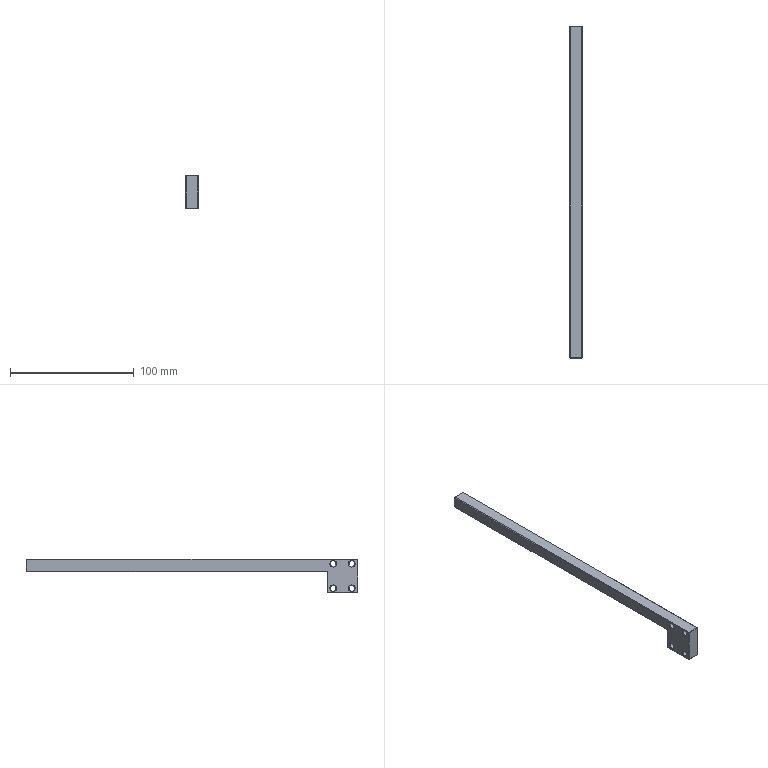Component | SolidWorks | BearingHousingAssembly-1_CylinderJaw1-1 | 1 solid | 60 faces | box 10 x 268 x 27 mm | volume 30124 mm3 | plane 32 | cone 18 | cylinder 10 | commonest cylinder face diameters 4.5 x8 3.3 x2 | material Plain Carbon Steel
build123d program:
from build123d import *

# Parameters (mm, degrees)
BOSS_EXTRUDE1_DEPTH            = 5
F_4_5_4_5_DIAMETER_HOLE1_D     = 4.5
F_4_5_4_5_DIAMETER_HOLE1_DEPTH = 50
F_4_5_4_5_DIAMETER_HOLE1_TIP   = 1.352
CHAMFER1_SIZE                  = 0.5
M4_TAPPED_HOLE1_D              = 3.3
M4_TAPPED_HOLE1_DEPTH          = 14
M4_TAPPED_HOLE1_TIP            = 0.9914


with BuildPart() as part:
    # Sketch1 → Boss-Extrude1 (new, symmetric)
    with BuildSketch(Plane.XY):
        Polygon((0, 0), (0, 268), (10, 268), (10, 25), (27, 25), (27, 0), align=None)
    extrude(amount=BOSS_EXTRUDE1_DEPTH, both=True)

    # 4.5 _4.5_ Diameter Hole1
    with Locations(Plane.XY.offset(5)):
        with Locations((3.5, 20), (23.5, 20), (23.5, 5), (3.5, 5)):
            Hole(F_4_5_4_5_DIAMETER_HOLE1_D / 2, depth=F_4_5_4_5_DIAMETER_HOLE1_DEPTH)
            with Locations((0, 0, -(F_4_5_4_5_DIAMETER_HOLE1_DEPTH + F_4_5_4_5_DIAMETER_HOLE1_TIP / 2))):  # 118° drill point
                Cone(0, F_4_5_4_5_DIAMETER_HOLE1_D / 2, F_4_5_4_5_DIAMETER_HOLE1_TIP, mode=Mode.SUBTRACT)

    # Chamfer1
    chamfer1_edges = [part.edges().sort_by_distance(p)[0] for p in [
        (18.5, 25, 5),
        (0, 0, 0),
        (0, 268, 0),
        (27, 25, 0),
        (27, 0, 0),
        (10, 146.5, 5),
        (5, 268, 5),
        (0, 134, 5),
        (5.75, 5, -5),
        (5.75, 5, 5),
        (25.75, 5, -5),
        (25.75, 5, 5),
        (25.75, 20, -5),
        (25.75, 20, 5),
        (13.5, 0, 5),
        (5.75, 20, -5),
        (5.75, 20, 5),
        (0, 134, -5),
        (5, 268, -5),
        (10, 146.5, -5),
        (27, 12.5, 5),
        (18.5, 25, -5),
        (27, 12.5, -5),
        (13.5, 0, -5),
    ]]
    chamfer(chamfer1_edges, length=CHAMFER1_SIZE)

    # M4 Tapped Hole1
    with Locations(Plane(origin=(0, 268, 0), x_dir=(1, 0, 0), z_dir=(0, 1, 0))):
        with Locations((5, 0)):
            Hole(M4_TAPPED_HOLE1_D / 2, depth=M4_TAPPED_HOLE1_DEPTH)
            with Locations((0, 0, -(M4_TAPPED_HOLE1_DEPTH + M4_TAPPED_HOLE1_TIP / 2))):  # 118° drill point
                Cone(0, M4_TAPPED_HOLE1_D / 2, M4_TAPPED_HOLE1_TIP, mode=Mode.SUBTRACT)


solid = part.part

# Placed as in the assembly
solid = solid.moved(Location((-38.666, 81.464, -6), (0, 90, 0)))